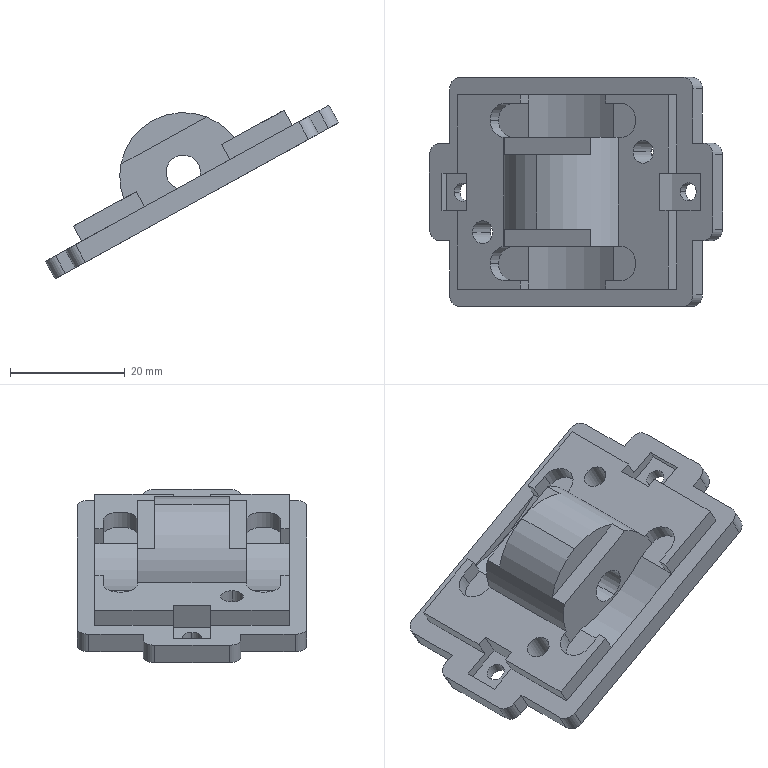Component | SolidWorks | Interrupteur haut-1 | 1 solid | 88 faces | box 51.18 x 40 x 30.31 mm | volume 10440 mm3 | plane 56 | cylinder 32 | commonest cylinder face diameters 4 x12 6 x10 3.2 x4 17.509 x2 22.237 x2 49.82 x2